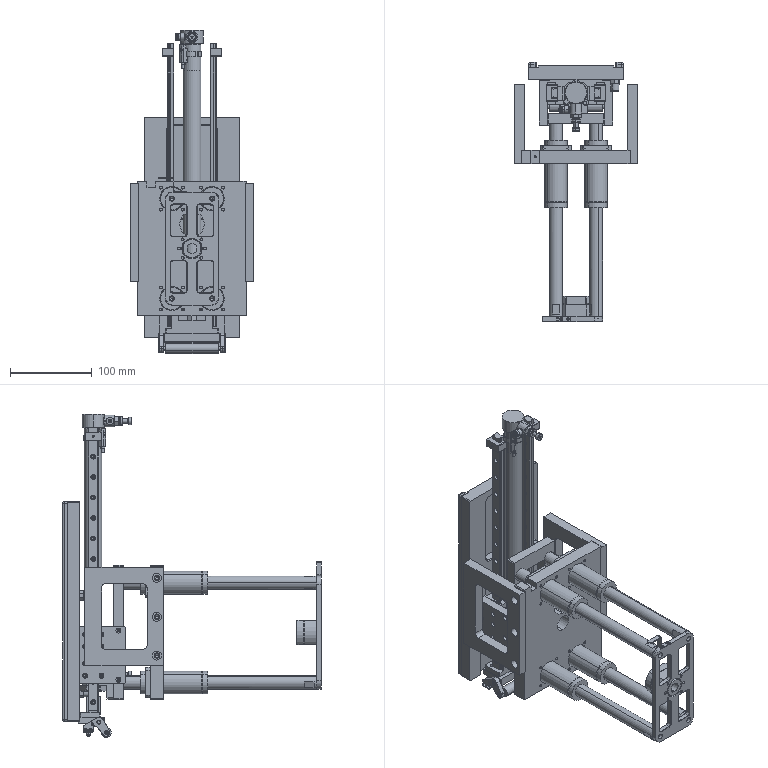Assembly | SolidWorks | mm | 61 component files | 62 solids | 3422 faces | box 150 x 316.25 x 394.73 mm | volume 1627100 mm3 | plane 1439 | cylinder 1289 | cone 438 | spline 214 | torus 24 | sphere 18 | commonest cylinder face diameters 6 x162 5 x106 3.4 x100 4 x84 2.5 x62 4.5 x60 3 x60 3.3 x48
Bill of materials:
ElasticPIN5N- | 3 |  | Stepped revolved part: a smaller-diameter hollow tube on top, a thin circular flange, a larger-diameter cylindrical body with a rounded lower end, and a short small-diameter boss at the bottom.
F01AE00111-A2007 | 1 | 6061 Alloy | Rectangular block with two parallel elongated through slots near the ends of its large face, chamfered corners, and a stepped/relieved end region with one larger and one smaller hole in the end face.
F01AE00111-A2008 | 2 | AISI 304 | Solid stepped cylindrical pin with two coaxial diameters: a shorter, smaller-diameter section and a longer, larger-diameter section, with small edge chamfers.
F01AE00111-A2010 | 1 | AISI 304 | Flat, constant-thickness bent-shaped link plate (boomerang/L outline) with rounded ends, two large through holes, two smaller through holes, an angled obround slot, and a rounded internal notch.
F01AE00111-A2011 | 1 | 6061 Alloy | Long rectangular bar with three evenly spaced through holes along its length, two U-shaped open notches at the ends of one long edge, rounded corners along one long edge, and two small holes in one end face.
F01AE00111-A2013 | 1 | AISI 304 | Flat bent-shaped link plate with the same general outline as unnamed part, but with counterbores or recessed rings around the two large holes; it also has two smaller holes, an angled obround slot, and a rounded internal notch.
F01AE00111-A2140 | 1 | AISI 304 | Long cylindrical roller- or shaft-like body with stepped, reduced-diameter journals at both ends; each journal has an intermediate shoulder step, and the visible end has a small axial hole.
L-740zz- | 8 |  | Plain annular ring (spacer/bushing-like) with a cylindrical outer surface, a concentric through bore, and flat parallel faces.
PIN 2X15- | 2 |  | Plain solid cylindrical rod or pin with chamfered ends.
F01AE00111-A2051 | 2 |  | Thick rectangular plate with an array of 13 round through holes and stepped lips along two opposite edges on the back side (a C-shaped edge profile).
F01AE00111-A2052 | 1 |  | Large rectangular plate with two shallow rounded-rectangle pockets on one face, several small holes in rows beside the pockets, holes in a narrow edge, and a raised step/land along one face.
F01AE00111-A2053 | 2 |  | Long, thin, narrow flat strip with seven evenly spaced small holes or short slots along its length and rounded ends or corners.
F01AE00111-A2055 | 1 |  | L-shaped bracket: a horizontal plate with one large round through-hole, joined to a shorter vertical leg that has two small through-holes.
F01AE00111-A2056 | 1 |  | Rectangular base plate with two upright stepped walls, one near each end. The base has a central through-hole and two end holes; each wall has a small hole.
F01AE00111-A2203 | 2 |  | U- or C-shaped channel block with one small through-hole in the back wall.
KJH06-M5 | 2 |  | Round fitting-like body along one axis: a cylindrical sleeve with a groove near one end, a hexagonal section, and a smaller chamfered spigot. It has an axial through-bore.
MGN12CGuide280 | 2 |  | Long, thin straight bar with a row of evenly spaced small holes along its length. Its end profile is roughly rectangular with chamfered corners, two opposite semicircular grooves and a small side notch.
MGN12C-Slider | 4 |  | Stepped rectangular block with a lengthwise channel open on one side. The channel corners have semicircular grooves, the outer faces have shallow flange steps, and there is one small hole on the top face.
PSL401A | 2 |  | T-shaped round body. The main cylinder has a hex section, a smaller spigot at one end, and a stem at the other end with collars and a round knob-like head. A side branch carries a cylindrical port with a flanged lip.
F01AE00111-A2006 | 1 |  | Rectangular frame plate with a large rounded-rectangle central window. It has four counterbored holes around the window, two small holes near one end, and small holes in one narrow edge.
F01AE00111-A2014 | 4 | Hard Chrome Plated Rod | Square-ish flat plate with a large rounded-rectangle window and three through-holes along one edge. A step or rabbet reduces the thickness at one end.
F01AE00111-A2015 | 2 |  | Slender solid cylindrical rod or pin with chamfered ends. One end has a small axial center hole, and there is a short flat or slot feature near that end.
F01AE00111-A2016 | 1 |  | Thick rectangular plate with five large round holes (four arranged in pairs, each with four small surrounding holes) and one smaller round hole. It has stepped side edges, a small notch on the top edge, and small holes in the edge faces.
F01AE00111-A2019 | 1 |  | Rounded-corner rectangular flat plate with four corner holes and four rounded-rectangular windows. A central circular hole is surrounded by six small holes in a circular pattern, and there are two small holes in one edge face.
F01AE00111-A2020 | 1 |  | Flat strip of constant thickness bent into a Z (joggle) shape. It has two parallel end legs pointing opposite ways, joined by a perpendicular middle section through two radiused bends. One end leg has two round through-holes in a row. All strip corners are rounded.
F01AE00111-A2085 | 1 | 6061 Alloy | Thick ring-shaped block with a large central round bore. The outer edge is round with two parallel flats cut on opposite sides. Six round through-holes are spaced around the bore, three near each flat side. The faces are flat and parallel.
LHFSW-MX16- | 4 |  | Long hollow round tube with a square flange near one end. The flange has its corners chamfered off and four round through-holes, one at each corner. A short round boss sticks out past the flange on the far side. A through-bore runs the full length. There are small circular grooves or steps near each end of the tube.
SFS01205Nut- | 1 |  | Flanged round body with a central through-bore. The flange is round with two parallel flats and has six round through-holes in a circle around the hub. On one side of the flange is a cylindrical hub that is narrower than the flange and longer than the flange is thick. Both the hub end and the flange edges are chamfered.
Mates:
1. concentric | LHFSW-MX16--2 face at (-84.852, -19.502, -211.475) dir (0, -1, 0) r 14 | F01AE00111-A2014-1 face at (-84.852, 47.548, -211.475) dir (0, -1, 0) r 8
2. concentric | LHFSW-MX16--3 face at (-133.852, -19.502, -211.475) dir (0, -1, 0) r 14 | F01AE00111-A2014-3 face at (-133.852, 47.548, -211.475) dir (0, -1, 0) r 8
3. coincident | F01AE00111-A2014-1 face at (-84.852, -192.452, -211.475) dir (0, -1, 0) | F01AE00111-A2014-3 face at (-133.852, -192.452, -211.475) dir (0, -1, 0)
4. coincident | F01AE00111-A2014-2 face at (-133.852, -192.452, -333.475) dir (0, -1, 0) | F01AE00111-A2014-4 face at (-84.852, -192.452, -333.475) dir (0, -1, 0)
5. concentric | F01AE00111-A2016-1 face at (-133.852, -3.452, -333.475) dir (0, 1, 0) r 14 | LHFSW-MX16--6 face at (-133.852, -19.502, -333.475) dir (0, -1, 0) r 14
6. concentric | F01AE00111-A2016-1 face at (-84.852, -3.452, -333.475) dir (0, 1, 0) r 14 | LHFSW-MX16--5 face at (-84.852, -19.502, -333.475) dir (0, -1, 0) r 14
7. concentric | F01AE00111-A2016-1 face at (-120.417, 12.548, -346.91) dir (0, 1, 0) r 1.65 | LHFSW-MX16--6 face at (-120.417, 16.498, -346.91) dir (0, -1, 0) r 3.75
8. coincident | F01AE00111-A2016-1 face at (-109.352, 12.548, -272.475) dir (0, 1, 0) | LHFSW-MX16--6 face at (-120.594, 12.548, -320.217) dir (0, -1, 0)
9. concentric | F01AE00111-A2016-1 face at (-98.287, 12.548, -346.91) dir (0, 1, 0) r 1.65 | LHFSW-MX16--5 face at (-98.287, 16.498, -346.91) dir (0, -1, 0) r 3.75
10. coincident | F01AE00111-A2016-1 face at (-109.352, 12.548, -272.475) dir (0, 1, 0) | LHFSW-MX16--5 face at (-71.594, 12.548, -320.217) dir (0, -1, 0)
11. coincident | F01AE00111-A2014-1 face at (-84.852, -192.452, -211.475) dir (0, -1, 0) | F01AE00111-A2014-3 face at (-133.852, -192.452, -211.475) dir (0, -1, 0)
12. coincident | F01AE00111-A2014-3 face at (-133.852, -192.452, -211.475) dir (0, -1, 0) | F01AE00111-A2014-4 face at (-84.852, -192.452, -333.475) dir (0, -1, 0)
13. concentric | F01AE00111-A2014-3 face at (-133.852, 47.548, -211.475) dir (0, -1, 0) r 8 | F01AE00111-A2006-2 face at (-133.852, 57.548, -211.475) dir (0, 1, 0) r 2.75
14. concentric | F01AE00111-A2014-2 face at (-133.852, 47.548, -333.475) dir (0, -1, 0) r 8 | F01AE00111-A2006-2 face at (-133.852, 57.548, -333.475) dir (0, 1, 0) r 2.75
15. concentric | F01AE00111-A2014-2 face at (-133.852, 47.548, -333.475) dir (0, -1, 0) r 8 | LHFSW-MX16--6 face at (-133.852, -19.502, -333.475) dir (0, -1, 0) r 14
16. concentric | F01AE00111-A2014-4 face at (-84.852, 47.548, -333.475) dir (0, -1, 0) r 8 | F01AE00111-A2006-2 face at (-84.852, 47.548, -333.475) dir (0, -1, 0) r 6
17. concentric | F01AE00111-A2014-4 face at (-84.852, 47.548, -333.475) dir (0, -1, 0) r 8 | LHFSW-MX16--5 face at (-84.852, -19.502, -333.475) dir (0, -1, 0) r 14
18. concentric | LHFSW-MX16--2 face at (-84.852, -19.502, -211.475) dir (0, -1, 0) r 14 | F01AE00111-A2016-1 face at (-84.852, -3.452, -211.475) dir (0, 1, 0) r 14
19. coincident | F01AE00111-A2014-3 face at (-133.852, 45.548, -211.475) dir (0, 1, 0) | F01AE00111-A2006-2 face at (-109.352, 45.548, -272.475) dir (0, -1, 0)
20. concentric | LHFSW-MX16--2 face at (-98.287, 16.498, -198.04) dir (0, -1, 0) r 3.75 | F01AE00111-A2016-1 face at (-98.287, 12.548, -198.04) dir (0, 1, 0) r 1.65
21. concentric | LHFSW-MX16--3 face at (-120.417, 16.498, -198.04) dir (0, -1, 0) r 3.75 | F01AE00111-A2016-1 face at (-120.417, 12.548, -198.04) dir (0, 1, 0) r 1.65
22. coincident | LHFSW-MX16--2 face at (-71.594, 12.548, -198.217) dir (0, -1, 0) | F01AE00111-A2016-1 face at (-109.352, 12.548, -272.475) dir (0, 1, 0)
23. coincident | LHFSW-MX16--3 face at (-120.594, 12.548, -198.217) dir (0, -1, 0) | F01AE00111-A2016-1 face at (-109.352, 12.548, -272.475) dir (0, 1, 0)
24. concentric | F01AE00111-A2016-1 face at (-42.352, 4.548, -252.975) dir (1, 0, 0) r 2.5 | F01AE00111-A2015-1 face at (-34.352, 4.548, -252.975) dir (1, 0, 0) r 5.5
25. concentric | F01AE00111-A2016-1 face at (-42.352, 4.548, -300.475) dir (1, 0, 0) r 2.5 | F01AE00111-A2015-1 face at (-34.352, 4.548, -300.475) dir (1, 0, 0) r 5.5
26. coincident | F01AE00111-A2015-1 face at (-44.352, 44.548, -252.975) dir (-1, 0, 0) | F01AE00111-A2016-1 face at (-44.352, -3.452, -272.475) dir (1, 0, 0)
27. concentric | F01AE00111-A2016-1 face at (-176.352, 4.548, -205.475) dir (-1, 0, 0) r 2.5 | F01AE00111-A2015-2 face at (-184.352, 4.548, -205.475) dir (-1, 0, 0) r 5.5
28. concentric | F01AE00111-A2016-1 face at (-176.352, 4.548, -252.975) dir (-1, 0, 0) r 2.5 | F01AE00111-A2015-2 face at (-184.352, 4.548, -252.975) dir (-1, 0, 0) r 5.5
29. coincident | F01AE00111-A2016-1 face at (-174.352, -3.452, -272.475) dir (-1, 0, 0) | F01AE00111-A2015-2 face at (-174.352, 44.548, -252.975) dir (1, 0, 0)
30. concentric | F01AE00111-A2014-1 face at (-84.852, -192.452, -211.475) dir (0, -1, 0) r 2.5 | F01AE00111-A2019-1 face at (-84.852, -196.452, -211.475) dir (0, 1, 0) r 3.25
31. concentric | F01AE00111-A2014-3 face at (-133.852, -192.452, -211.475) dir (0, -1, 0) r 2.5 | F01AE00111-A2019-1 face at (-133.852, -196.452, -211.475) dir (0, 1, 0) r 3.25
32. distance | F01AE00111-A2014-3 face at (-133.852, -192.452, -211.475) dir (0, -1, 0) | F01AE00111-A2019-1 face at (-133.852, -190.452, -211.475) dir (0, 1, 0)
33. coincident | F01AE00111-A2006-2 face at (-109.352, 57.548, -272.475) dir (0, 1, 0) | F01AE00111-A2000-21TopEdgeAssembly-1/F01AE00111-A2055-1 face at (-123.852, 57.548, -331.975) dir (0, -1, 0)
34. width | F01AE00111-A2000-21TopEdgeAssembly-1/F01AE00111-A2051-1 face at (-64.352, 72.173, -299.975) dir (1, 0, 0) | F01AE00111-A2000-21TopEdgeAssembly-1/F01AE00111-A2051-2 face at (-154.352, 72.173, -299.975) dir (-1, 0, 0) | F01AE00111-A2006-2 face at (-144.352, 57.548, -190.475) dir (-1, 0, 0) | F01AE00111-A2006-2 face at (-74.352, 57.548, -190.475) dir (1, 0, 0)
35. distance | F01AE00111-A2016-1 face at (-109.352, 12.548, -272.475) dir (0, 1, 0) | F01AE00111-A2006-2 face at (-109.352, 45.548, -272.475) dir (0, -1, 0)
36. coincident | F01AE00111-A2019-1 face at (-141.852, -196.452, -203.475) dir (0, 0, 1) | F01AE00111-A2020-1 face at (-116.352, -196.452, -203.475) dir (0, 0, -1)
37. concentric | F01AE00111-A2019-1 face at (-127.352, -193.452, -203.475) dir (0, 0, 1) r 1.25 | F01AE00111-A2020-1 face at (-127.352, -193.452, -203.475) dir (0, 0, 1) r 1.6
38. concentric | F01AE00111-A2019-1 face at (-119.352, -193.452, -203.475) dir (0, 0, 1) r 1.25 | F01AE00111-A2020-1 face at (-119.352, -193.452, -203.475) dir (0, 0, 1) r 1.6
39. concentric | F01AE00111-A2019-1 face at (-109.352, -196.452, -272.475) dir (0, 1, 0) r 12 | SFS01205Nut--1 face at (-109.352, -196.452, -272.475) dir (0, -1, 0) r 12
40. coincident | F01AE00111-A2019-1 face at (-133.852, -196.452, -211.475) dir (0, -1, 0) | SFS01205Nut--1 face at (-109.352, -196.452, -284.475) dir (0, -1, 0)
41. parallel | F01AE00111-A2019-1 face at (-141.852, -196.452, -203.475) dir (0, 0, 1) | SFS01205Nut--1 face at (-96.123, -46.07, -257.475) dir (0, 0, 1)
42. coincident | F01AE00111-A2019-1 face at (-133.852, -190.452, -211.475) dir (0, 1, 0) | F01AE00111-A2085-1 face at (-109.352, -190.452, -272.475) dir (0, -1, 0)
43. concentric | SFS01205Nut--1 face at (-109.352, -196.452, -272.475) dir (0, -1, 0) r 12 | F01AE00111-A2085-1 face at (-109.352, -175.452, -272.475) dir (0, -1, 0) r 20
44. coincident | SFS01205Nut--1 face at (-96.123, -46.07, -257.475) dir (0, 0, 1) | F01AE00111-A2085-1 face at (-96.123, -102.298, -257.475) dir (0, 0, 1)
45. concentric | F01AE00111-A2006-2 face at (-144.352, 51.548, -329.975) dir (-1, 0, 0) r 1.25 | F01AE00111-A2000-21TopEdgeAssembly-1/F01AE00111-A2051-2 face at (-154.352, 51.548, -329.975) dir (-1, 0, 0) r 1.7
46. coincident | F01AE00111-A2052-1 face at (-138.995, 246.366, -247.995) dir (0, 1, 0) | F01AE00111-A2053-1 face at (-191.995, 246.366, -247.995) dir (0, -1, 0)
47. coincident | F01AE00111-A2052-1 face at (-197.495, 248.366, -382.245) dir (0, 0, -1) | F01AE00111-A2053-1 face at (-196.995, 252.366, -382.245) dir (0, 0, -1)
48. distance | F01AE00111-A2053-1 face at (-186.995, 252.366, -113.745) dir (1, 0, 0) | F01AE00111-A2052-1 face at (-184.995, 246.366, -382.245) dir (-1, 0, 0)
49. coincident | F01AE00111-A2052-1 face at (-138.995, 246.366, -247.995) dir (0, 1, 0) | F01AE00111-A2053-2 face at (-85.995, 246.366, -247.995) dir (0, -1, 0)
50. coincident | F01AE00111-A2052-1 face at (-197.495, 248.366, -382.245) dir (0, 0, -1) | F01AE00111-A2053-2 face at (-80.995, 252.366, -382.245) dir (0, 0, -1)
51. distance | F01AE00111-A2052-1 face at (-92.995, 246.366, -382.245) dir (1, 0, 0) | F01AE00111-A2053-2 face at (-90.995, 252.366, -382.245) dir (-1, 0, 0)
52. coincident | F01AE00111-A2051-1 face at (-93.995, 178.116, -336.245) dir (0, 0, -1) | F01AE00111-A2051-2 face at (-183.995, 178.116, -336.245) dir (0, 0, -1)
53. coincident | F01AE00111-A2052-1 face at (-138.995, 231.366, -247.995) dir (0, -1, 0) | KJH06-M5-2 face at (-94.749, 231.366, -349.371) dir (0, 1, 0)
54. concentric | F01AE00111-A2052-1 face at (-91.495, 231.366, -347.245) dir (0, -1, 0) r 2.1 | KJH06-M5-2 face at (-91.495, 222.516, -347.245) dir (0, 1, 0) r 5
55. coincident | F01AE00111-A2052-1 face at (-138.995, 231.366, -247.995) dir (0, -1, 0) | KJH06-M5-1 face at (-94.749, 231.366, -230.371) dir (0, 1, 0)
56. concentric | F01AE00111-A2052-1 face at (-91.495, 231.366, -228.245) dir (0, -1, 0) r 2.1 | KJH06-M5-1 face at (-91.495, 222.516, -228.245) dir (0, 1, 0) r 5
57. coincident | F01AE00111-A2051-1 face at (-93.995, 231.366, -266.245) dir (0, 1, 0) | F01AE00111-A2051-2 face at (-183.995, 231.366, -336.245) dir (0, 1, 0)
58. coincident | F01AE00111-A2051-1 face at (-93.995, 178.116, -336.245) dir (0, 0, -1) | F01AE00111-A2051-2 face at (-183.995, 178.116, -336.245) dir (0, 0, -1)
59. distance | F01AE00111-A2055-1 face at (-176.905, 190.116, -355.245) dir (0, 0, -1) | F01AE00111-A2052-1 face at (-197.495, 248.366, -382.245) dir (0, 0, -1)
60. width | F01AE00111-A2055-1 face at (-124.495, 190.116, -333.245) dir (1, 0, 0) | F01AE00111-A2055-1 face at (-153.495, 190.116, -333.245) dir (-1, 0, 0) | F01AE00111-A2051-1 face at (-93.995, 204.741, -301.245) dir (1, 0, 0) | F01AE00111-A2051-2 face at (-183.995, 204.741, -301.245) dir (-1, 0, 0)
61. coincident | F01AE00111-A2052-1 face at (-138.995, 231.366, -247.995) dir (0, -1, 0) | F01AE00111-A2051-2 face at (-183.995, 231.366, -336.245) dir (0, 1, 0)
62. parallel | F01AE00111-A2051-2 face at (-183.995, 231.366, -336.245) dir (0, 1, 0) | F01AE00111-A2056-1 face at (-178.995, 223.366, -371.245) dir (0, 1, 0)
63. width | F01AE00111-A2056-1 face at (-116.995, 208.866, -383.614) dir (1, 0, 0) | F01AE00111-A2056-1 face at (-160.995, 220.866, -383.614) dir (-1, 0, 0) | F01AE00111-A2055-1 face at (-153.495, 190.116, -333.245) dir (-1, 0, 0) | F01AE00111-A2055-1 face at (-124.495, 190.116, -333.245) dir (1, 0, 0)
64. coincident | F01AE00111-A2056-1 face at (-171.495, 231.366, -377.245) dir (0, 0, -1) | F01AE00111-A2000-19TopEdgeRollerAssembly-1/F01AE00111-A2007-1 face at (-138.995, 216.366, -377.245) dir (0, 0, 1)
65. width | F01AE00111-A2000-19TopEdgeRollerAssembly-1/F01AE00111-A2007-1 face at (-104.995, 201.366, -387.245) dir (1, 0, 0) | F01AE00111-A2000-19TopEdgeRollerAssembly-1/F01AE00111-A2007-1 face at (-172.995, 201.366, -387.245) dir (-1, 0, 0) | F01AE00111-A2056-1 face at (-171.495, 231.366, -371.245) dir (-1, 0, 0) | F01AE00111-A2056-1 face at (-106.495, 231.366, -377.245) dir (1, 0, 0)
66. distance | F01AE00111-A2000-19TopEdgeRollerAssembly-1/F01AE00111-A2007-1 face at (-77.495, 233.366, -387.245) dir (0, 1, 0) | F01AE00111-A2056-1 face at (-138.995, 231.366, -377.245) dir (0, 1, 0)
67. coincident | F01AE00111-A2056-1 face at (-116.995, 208.866, -383.614) dir (1, 0, 0) | MGN12CGuide280-1 face at (-116.995, 216.666, -368.745) dir (-1, 0, 0)
68. concentric | F01AE00111-A2056-1 face at (-116.995, 214.866, -358.745) dir (1, 0, 0) r 1.25 | MGN12CGuide280-1 edge at (-112.495, 214.866, -358.745) dir (1, 0, 0) r 3
69. parallel | F01AE00111-A2056-1 face at (-138.995, 206.366, -377.245) dir (0, -1, 0) | MGN12CGuide280-1 face at (-112.745, 208.866, -368.745) dir (0, -1, 0)
70. coincident | F01AE00111-A2056-1 face at (-160.995, 220.866, -383.614) dir (-1, 0, 0) | MGN12CGuide280-2 face at (-160.995, 220.866, -368.745) dir (1, 0, 0)
71. concentric | F01AE00111-A2056-1 face at (-160.995, 214.866, -358.745) dir (-1, 0, 0) r 1.25 | MGN12CGuide280-2 face at (-152.018, 214.866, -358.745) dir (1, 0, 0) r 1.75
72. parallel | F01AE00111-A2056-1 face at (-138.995, 206.366, -377.245) dir (0, -1, 0) | MGN12CGuide280-2 face at (-160.995, 208.866, -368.745) dir (0, -1, 0)
73. coincident | MGN12C-Slider-1 face at (-173.995, 201.366, -301.545) dir (-1, 0, 0) | MGN12C-Slider-2 face at (-173.995, 201.366, -266.245) dir (-1, 0, 0)
74. coincident | MGN12C-Slider-1 face at (-173.995, 228.366, -301.545) dir (0, 1, 0) | MGN12C-Slider-2 face at (-173.995, 228.366, -266.245) dir (0, 1, 0)
75. distance | MGN12C-Slider-1 face at (-166.995, 228.366, -336.245) dir (0, 0, -1) | MGN12C-Slider-2 face at (-166.995, 228.366, -266.245) dir (0, 0, 1)
76. concentric | MGN12C-Slider-2 face at (-166.495, 220.866, -248.595) dir (0, 0, -1) r 1.25 | MGN12CGuide280-2 face at (-166.495, 220.866, -368.745) dir (0, 0, 1) r 1.25
77. concentric | MGN12C-Slider-2 face at (-166.495, 208.866, -248.595) dir (0, 0, -1) r 1.25 | MGN12CGuide280-2 face at (-166.495, 208.866, -368.745) dir (0, 0, 1) r 1.25
78. coincident | F01AE00111-A2051-2 face at (-183.995, 178.116, -336.245) dir (0, 0, -1) | MGN12C-Slider-1 face at (-166.995, 228.366, -336.245) dir (0, 0, -1)
79. coincident | MGN12C-Slider-3 face at (-103.995, 228.366, -301.545) dir (1, 0, 0) | MGN12C-Slider-4 face at (-103.995, 228.366, -266.245) dir (1, 0, 0)
80. coincident | MGN12C-Slider-3 face at (-103.995, 201.366, -301.545) dir (0, -1, 0) | MGN12C-Slider-4 face at (-103.995, 201.366, -266.245) dir (0, -1, 0)
81. distance | MGN12C-Slider-3 face at (-110.995, 201.366, -336.245) dir (0, 0, -1) | MGN12C-Slider-4 face at (-110.995, 201.366, -266.245) dir (0, 0, 1)
82. concentric | MGN12CGuide280-1 face at (-111.495, 220.866, -368.745) dir (0, 0, 1) r 1.25 | MGN12C-Slider-3 face at (-111.495, 220.866, -283.895) dir (0, 0, -1) r 1.25
83. concentric | MGN12CGuide280-1 face at (-111.495, 208.866, -368.745) dir (0, 0, 1) r 1.25 | MGN12C-Slider-3 face at (-111.495, 208.866, -283.895) dir (0, 0, -1) r 1.25
84. coincident | F01AE00111-A2051-1 face at (-93.995, 178.116, -336.245) dir (0, 0, -1) | MGN12C-Slider-3 face at (-110.995, 201.366, -336.245) dir (0, 0, -1)
85. coincident | F01AE00111-A2051-2 face at (-173.995, 204.741, -301.245) dir (1, 0, 0) | MGN12C-Slider-1 face at (-173.995, 201.366, -301.545) dir (-1, 0, 0)
86. concentric | F01AE00111-A2055-1 face at (-138.995, 215.116, -329.245) dir (0, 0, -1) r 11.25 | MA20x250SU(0)+(CS1-M-2)-1/20MAU250 Body-1 face at (-138.995, 215.116, -7.245) dir (0, 0, -1) r 11
87. coincident | F01AE00111-A2055-1 face at (-138.995, 209.116, -333.245) dir (0, 0, 1) | MA20x250SU(0)+(CS1-M-2)-1/20MAU250 Body-1 face at (-138.995, 204.116, -333.245) dir (0, 0, -1)
88. coincident | F01AE00111-A2051-1 face at (-103.995, 228.366, -349.587) dir (0, -1, 0) | MGN12C-Slider-4 face at (-113.995, 228.366, -266.245) dir (0, 1, 0)
89. coincident | PSL401A-1 face at (-133.795, 179.266, -15.245) dir (0, -1, 0) | PSL401A-2 face at (-133.964, 179.266, -326.56) dir (0, -1, 0)
90. parallel | F01AE00111-A2055-1 face at (-153.495, 190.116, -333.245) dir (0, -1, 0) | PSL401A-2 face at (-135.029, 168.116, -326.282) dir (0, -1, 0)
91. concentric | F01AE00111-A2056-1 face at (-138.995, 215.116, -361.245) dir (0, 0, 1) r 3.4 | MA20x250SU(0)+(CS1-M-2)-1/20UMA250 Rod-1 face at (-138.995, 215.116, -34.245) dir (0, 0, -1) r 4
92. coincident | F01AE00111-A2056-1 face at (-154.995, 172.84, -361.245) dir (0, 0, 1) | MA20x250SU(0)+(CS1-M-2)-1/20 MA Nut1-1 face at (-138.995, 221.116, -361.245) dir (0, 0, -1)
93. concentric | F01AE00111-A2052-1 face at (-100.995, 231.366, -331.245) dir (0, 1, 0) r 1.75 | F01AE00111-A2051-1 face at (-100.995, 231.366, -331.245) dir (0, 1, 0) r 1.25
94. concentric | MGN12CGuide280-2 face at (-168.995, 214.866, -33.745) dir (-1, 0, 0) r 1.7 | F01AE00111-A2203-1 face at (-174.995, 214.866, -33.745) dir (-1, 0, 0) r 1.25
95. coincident | MGN12CGuide280-2 face at (-168.995, 208.866, -368.745) dir (-1, 0, 0) | F01AE00111-A2203-1 face at (-168.995, 221.366, -42.745) dir (1, 0, 0)
96. parallel | MGN12CGuide280-2 face at (-160.995, 213.366, -23.745) dir (0, 0, 1) | F01AE00111-A2203-1 face at (-174.995, 224.866, -28.745) dir (0, 0, 1)
97. concentric | MGN12CGuide280-1 face at (-108.995, 214.866, -33.745) dir (1, 0, 0) r 3 | F01AE00111-A2203-2 face at (-102.995, 214.866, -33.745) dir (1, 0, 0) r 1.25
98. coincident | MGN12CGuide280-1 face at (-108.995, 220.866, -368.745) dir (1, 0, 0) | F01AE00111-A2203-2 face at (-108.995, 208.366, -42.745) dir (-1, 0, 0)
99. parallel | MGN12CGuide280-1 face at (-116.995, 216.366, -23.745) dir (0, 0, 1) | F01AE00111-A2203-2 face at (-102.995, 204.866, -28.745) dir (0, 0, 1)
100. concentric | MA20x250SU(0)+(CS1-M-2)-1/20MAU250 Body-1 face at (-138.995, 212.116, -15.245) dir (0, 1, 0) r 4.864 | PSL401A-1 face at (-138.995, 168.116, -15.245) dir (0, 1, 0) r 4.864
101. coincident | MA20x250SU(0)+(CS1-M-2)-1/20MAU250 Body-1 edge at (-138.995, 209.616, -15.245) dir (0, 1, 0) r 4.283 | PSL401A-1 edge at (-138.995, 209.616, -15.245) dir (0, 1, 0) r 4.283
102. concentric | MA20x250SU(0)+(CS1-M-2)-1/20MAU250 Body-1 face at (-138.995, 212.116, -325.245) dir (0, 1, 0) r 4.864 | PSL401A-2 face at (-138.995, 168.116, -325.245) dir (0, 1, 0) r 4.864
103. coincident | F01AE00111-A2007-1 face at (-75.402, 7.5, -23.9) dir (0, -1, 0) | F01AE00111-A2008-1 face at (-74.302, 7.5, -21.655) dir (0, 1, 0)
104. concentric | F01AE00111-A2007-1 face at (-75.402, 6, -23.9) dir (0, -1, 0) r 2.5 | F01AE00111-A2008-1 face at (-75.402, 7.5, -23.9) dir (0, 1, 0) r 2.5
105. concentric | F01AE00111-A2007-1 face at (-76.902, -2, -15.4) dir (0, -1, 0) r 1 | PIN 2X15--1 face at (-76.902, -7, -15.4) dir (0, 1, 0) r 1
106. distance | PIN 2X15--1 face at (-76.902, -7, -15.4) dir (0, -1, 0) | F01AE00111-A2007-1 face at (-79.402, -2, -30.5) dir (0, -1, 0)
107. coincident | F01AE00111-A2007-1 face at (-75.402, 56.5, -23.9) dir (0, 1, 0) | F01AE00111-A2008-2 face at (-72.928, 56.5, -23.542) dir (0, -1, 0)
108. concentric | F01AE00111-A2007-1 face at (-75.402, 58, -23.9) dir (0, 1, 0) r 2.5 | F01AE00111-A2008-2 face at (-75.402, 56.5, -23.9) dir (0, -1, 0) r 2.5
109. concentric | F01AE00111-A2007-1 face at (-76.902, 66, -15.4) dir (0, 1, 0) r 1 | PIN 2X15--2 face at (-76.902, 56, -15.4) dir (0, 1, 0) r 1
110. distance | F01AE00111-A2007-1 face at (-79.402, 66, -30.5) dir (0, 1, 0) | PIN 2X15--2 face at (-76.902, 71, -15.4) dir (0, 1, 0)
111. coincident | F01AE00111-A2010-1 face at (-82.402, 66.5, -19.093) dir (0, -1, 0) | F01AE00111-A2011-1 face at (-88.402, 66.5, -4.89) dir (0, 1, 0)
112. concentric | F01AE00111-A2010-1 face at (-85.402, 72.5, -7.89) dir (0, 1, 0) r 2.5 | F01AE00111-A2011-1 face at (-85.402, 66.5, -7.89) dir (0, 1, 0) r 1.025
113. concentric | F01AE00111-A2010-1 face at (-85.402, 72.5, -13.89) dir (0, 1, 0) r 1.45 | F01AE00111-A2011-1 face at (-85.402, 66.5, -13.89) dir (0, 1, 0) r 1.025
114. coincident | F01AE00111-A2013-1 face at (-82.402, -2.5, -19.093) dir (0, 1, 0) | F01AE00111-A2011-1 face at (-88.402, -2.5, -4.89) dir (0, -1, 0)
115. concentric | F01AE00111-A2013-1 face at (-85.402, -8.5, -7.89) dir (0, -1, 0) r 2.5 | F01AE00111-A2011-1 face at (-85.402, -2.5, -7.89) dir (0, -1, 0) r 1.025
116. concentric | F01AE00111-A2013-1 face at (-85.402, -8.5, -13.89) dir (0, -1, 0) r 1.45 | F01AE00111-A2011-1 face at (-85.402, -2.5, -13.89) dir (0, -1, 0) r 1.025
117. coincident | L-740zz--1 face at (-75.402, -5, -23.9) dir (0, 1, 0) | L-740zz--2 face at (-75.402, -5, -23.9) dir (0, -1, 0)
118. concentric | L-740zz--1 face at (-75.402, -7.5, -23.9) dir (0, 1, 0) r 3.5 | L-740zz--2 face at (-75.402, -5, -23.9) dir (0, 1, 0) r 3.5
119. coincident | F01AE00111-A2013-1 face at (-75.402, -7.5, -23.9) dir (0, 1, 0) | L-740zz--1 face at (-75.402, -7.5, -23.9) dir (0, -1, 0)
120. concentric | F01AE00111-A2013-1 face at (-75.402, -7.5, -23.9) dir (0, 1, 0) r 3.5 | L-740zz--1 face at (-75.402, -7.5, -23.9) dir (0, 1, 0) r 3.5
121. coincident | L-740zz--3 face at (-88.13, -5, -32.812) dir (0, -1, 0) | L-740zz--6 face at (-88.13, -5, -32.812) dir (0, 1, 0)
122. concentric | L-740zz--3 face at (-88.13, -5, -32.812) dir (0, 1, 0) r 3.5 | L-740zz--6 face at (-88.13, -7.5, -32.812) dir (0, 1, 0) r 3.5
123. coincident | F01AE00111-A2013-1 face at (-88.13, -7.5, -32.812) dir (0, 1, 0) | L-740zz--6 face at (-88.13, -7.5, -32.812) dir (0, -1, 0)
124. concentric | F01AE00111-A2013-1 face at (-88.13, -7.5, -32.812) dir (0, 1, 0) r 3.5 | L-740zz--6 face at (-88.13, -7.5, -32.812) dir (0, 1, 0) r 3.5
125. coincident | F01AE00111-A2140-1 face at (-88.758, -2.5, -34.711) dir (0, -1, 0) | L-740zz--3 face at (-88.13, -2.5, -32.812) dir (0, 1, 0)
126. concentric | F01AE00111-A2140-1 face at (-88.13, -16.971, -32.812) dir (0, 1, 0) r 6 | L-740zz--3 face at (-88.13, -5, -32.812) dir (0, 1, 0) r 2
127. coincident | L-740zz--5 face at (-88.13, 69, -32.812) dir (0, -1, 0) | L-740zz--7 face at (-88.13, 69, -32.812) dir (0, 1, 0)
128. concentric | L-740zz--5 face at (-88.13, 69, -32.812) dir (0, 1, 0) r 3.5 | L-740zz--7 face at (-88.13, 66.5, -32.812) dir (0, 1, 0) r 3.5
129. coincident | F01AE00111-A2010-1 face at (-82.402, 66.5, -19.093) dir (0, -1, 0) | L-740zz--7 face at (-88.13, 66.5, -32.812) dir (0, -1, 0)
130. concentric | F01AE00111-A2010-1 face at (-88.13, 72.5, -32.812) dir (0, -1, 0) r 2.5 | L-740zz--7 face at (-88.13, 66.5, -32.812) dir (0, 1, 0) r 3.5
131. coincident | L-740zz--8 face at (-75.402, 69, -23.9) dir (0, -1, 0) | L-740zz--9 face at (-75.402, 69, -23.9) dir (0, 1, 0)
132. concentric | L-740zz--8 face at (-75.402, 69, -23.9) dir (0, 1, 0) r 3.5 | L-740zz--9 face at (-75.402, 66.5, -23.9) dir (0, 1, 0) r 3.5
133. concentric | F01AE00111-A2010-1 face at (-75.402, 71.5, -23.9) dir (0, -1, 0) r 3.5 | L-740zz--9 face at (-75.402, 66.5, -23.9) dir (0, 1, 0) r 2
134. coincident | F01AE00111-A2010-1 face at (-82.402, 66.5, -19.093) dir (0, -1, 0) | L-740zz--9 face at (-75.402, 66.5, -23.9) dir (0, -1, 0)
135. concentric | F01AE00111-A2008-1 face at (-75.402, 7.5, -23.9) dir (0, 1, 0) r 2 | L-740zz--1 face at (-75.402, -7.5, -23.9) dir (0, 1, 0) r 2
136. coincident | F01AE00111-A2008-1 face at (-74.522, -2.5, -22.104) dir (0, -1, 0) | F01AE00111-A2013-1 face at (-82.402, -2.5, -19.093) dir (0, 1, 0)
137. parallel | F01AE00111-A2007-1 face at (-79.402, 32, -15.5) dir (-1, 0, 0) | F01AE00111-A2011-1 face at (-88.402, 32, -10.89) dir (-1, 0, 0)
138. coincident | ElasticPIN5N--2 face at (-80.402, 32, -10.89) dir (-1, 0, 0) | ElasticPIN5N--3 face at (-80.402, 49.5, -10.89) dir (-1, 0, 0)
139. coincident | ElasticPIN5N--1 face at (-80.402, 14.5, -10.89) dir (-1, 0, 0) | ElasticPIN5N--2 face at (-80.402, 32, -10.89) dir (-1, 0, 0)
140. concentric | F01AE00111-A2011-1 face at (-82.402, 14.5, -10.89) dir (-1, 0, 0) r 2.5 | ElasticPIN5N--1 face at (-68.752, 14.5, -10.89) dir (-1, 0, 0) r 2.5
141. concentric | F01AE00111-A2011-1 face at (-82.402, 32, -10.89) dir (-1, 0, 0) r 2.5 | ElasticPIN5N--2 face at (-68.752, 32, -10.89) dir (-1, 0, 0) r 2.5
142. concentric | F01AE00111-A2011-1 face at (-82.402, 49.5, -10.89) dir (-1, 0, 0) r 2.5 | ElasticPIN5N--3 face at (-68.752, 49.5, -10.89) dir (-1, 0, 0) r 2.5
143. coincident | F01AE00111-A2011-1 face at (-80.402, 32, -10.89) dir (1, 0, 0) | ElasticPIN5N--1 face at (-80.402, 14.5, -10.89) dir (-1, 0, 0)
144. coincident | 20MAU250 Body-1 axis at (-108.9, 0, 0) dir (1, 0, 0) | 20UMA250 Rod-1 axis at (-136.9, 0, 0) dir (1, 0, 0)
145. angle | 20UMA250 Rod-1 plane at (-56, 0, 0) dir (0, 0, -1) | 20MAU250 Body-1 plane at (-28, 0, 0) dir (0, 0, -1)
146. coincident | 20MAU250 Body-1 axis at (-108.9, 0, 0) dir (1, 0, 0) | 20 MA Nut-1 axis at (-108.9, 0, 0) dir (1, 0, 0)
147. angle | 20 MA Nut-1 plane at (-28, 0, 0) dir (0, 0, -1) | 20MAU250 Body-1 plane at (-28, 0, 0) dir (0, 0, -1)
148. coincident | 20MAU250 Body-1 axis at (-108.9, 0, 0) dir (1, 0, 0) | 20 MA Nut1-1 axis at (39.9, 0, 0) dir (-1, 0, 0)
149. angle | 20 MA Nut1-1 plane at (-41, 0, 0) dir (0, 0, -1) | 20MAU250 Body-1 plane at (-28, 0, 0) dir (0, 0, -1)
150. distance | CS1-M-S20-1 plane at (1, 0, 0) dir (1, 0, 0) | 20MAU250 Body-1 plane at (1, 0, 0) dir (-1, 0, 0)
151. coincident | 20MAU250 Body-1 axis at (-108.9, 0, 0) dir (1, 0, 0) | CS1-M-S20-1 axis at (81.9, 0, 0) dir (-1, 0, 0)
152. angle | CS1-M-S20-1 plane at (1, 0, 0) dir (0, 0.7071, -0.7071) | 20MAU250 Body-1 plane at (-28, 0, 0) dir (0, 0, -1)
153. distance | CS1-M-S20-2 plane at (293, 0, 0) dir (-1, 0, 0) | 20MAU250 Body-1 plane at (293, 0, 0) dir (1, 0, 0)
154. coincident | 20MAU250 Body-1 axis at (52.9, 0, 0) dir (-1, 0, 0) | CS1-M-S20-2 axis at (212.1, 0, 0) dir (1, 0, 0)
155. angle | CS1-M-S20-2 plane at (293, 0, 0) dir (0, 0.7071, 0.7071) | 20MAU250 Body-1 plane at (-28, 0, 0) dir (0, 0, -1)
156. distance | 20UMA250 Rod-1 face at (-56, 0, 0) dir (-1, 0, 0) | 20MAU250 Body-1 face at (-28, 0, 0) dir (-1, 0, 0)
157. distance | 20UMA250 Rod-1 face at (-56, 0, 0) dir (-1, 0, 0) | 20 MA Nut1-1 face at (-44, -6, 0) dir (-1, 0, 0)